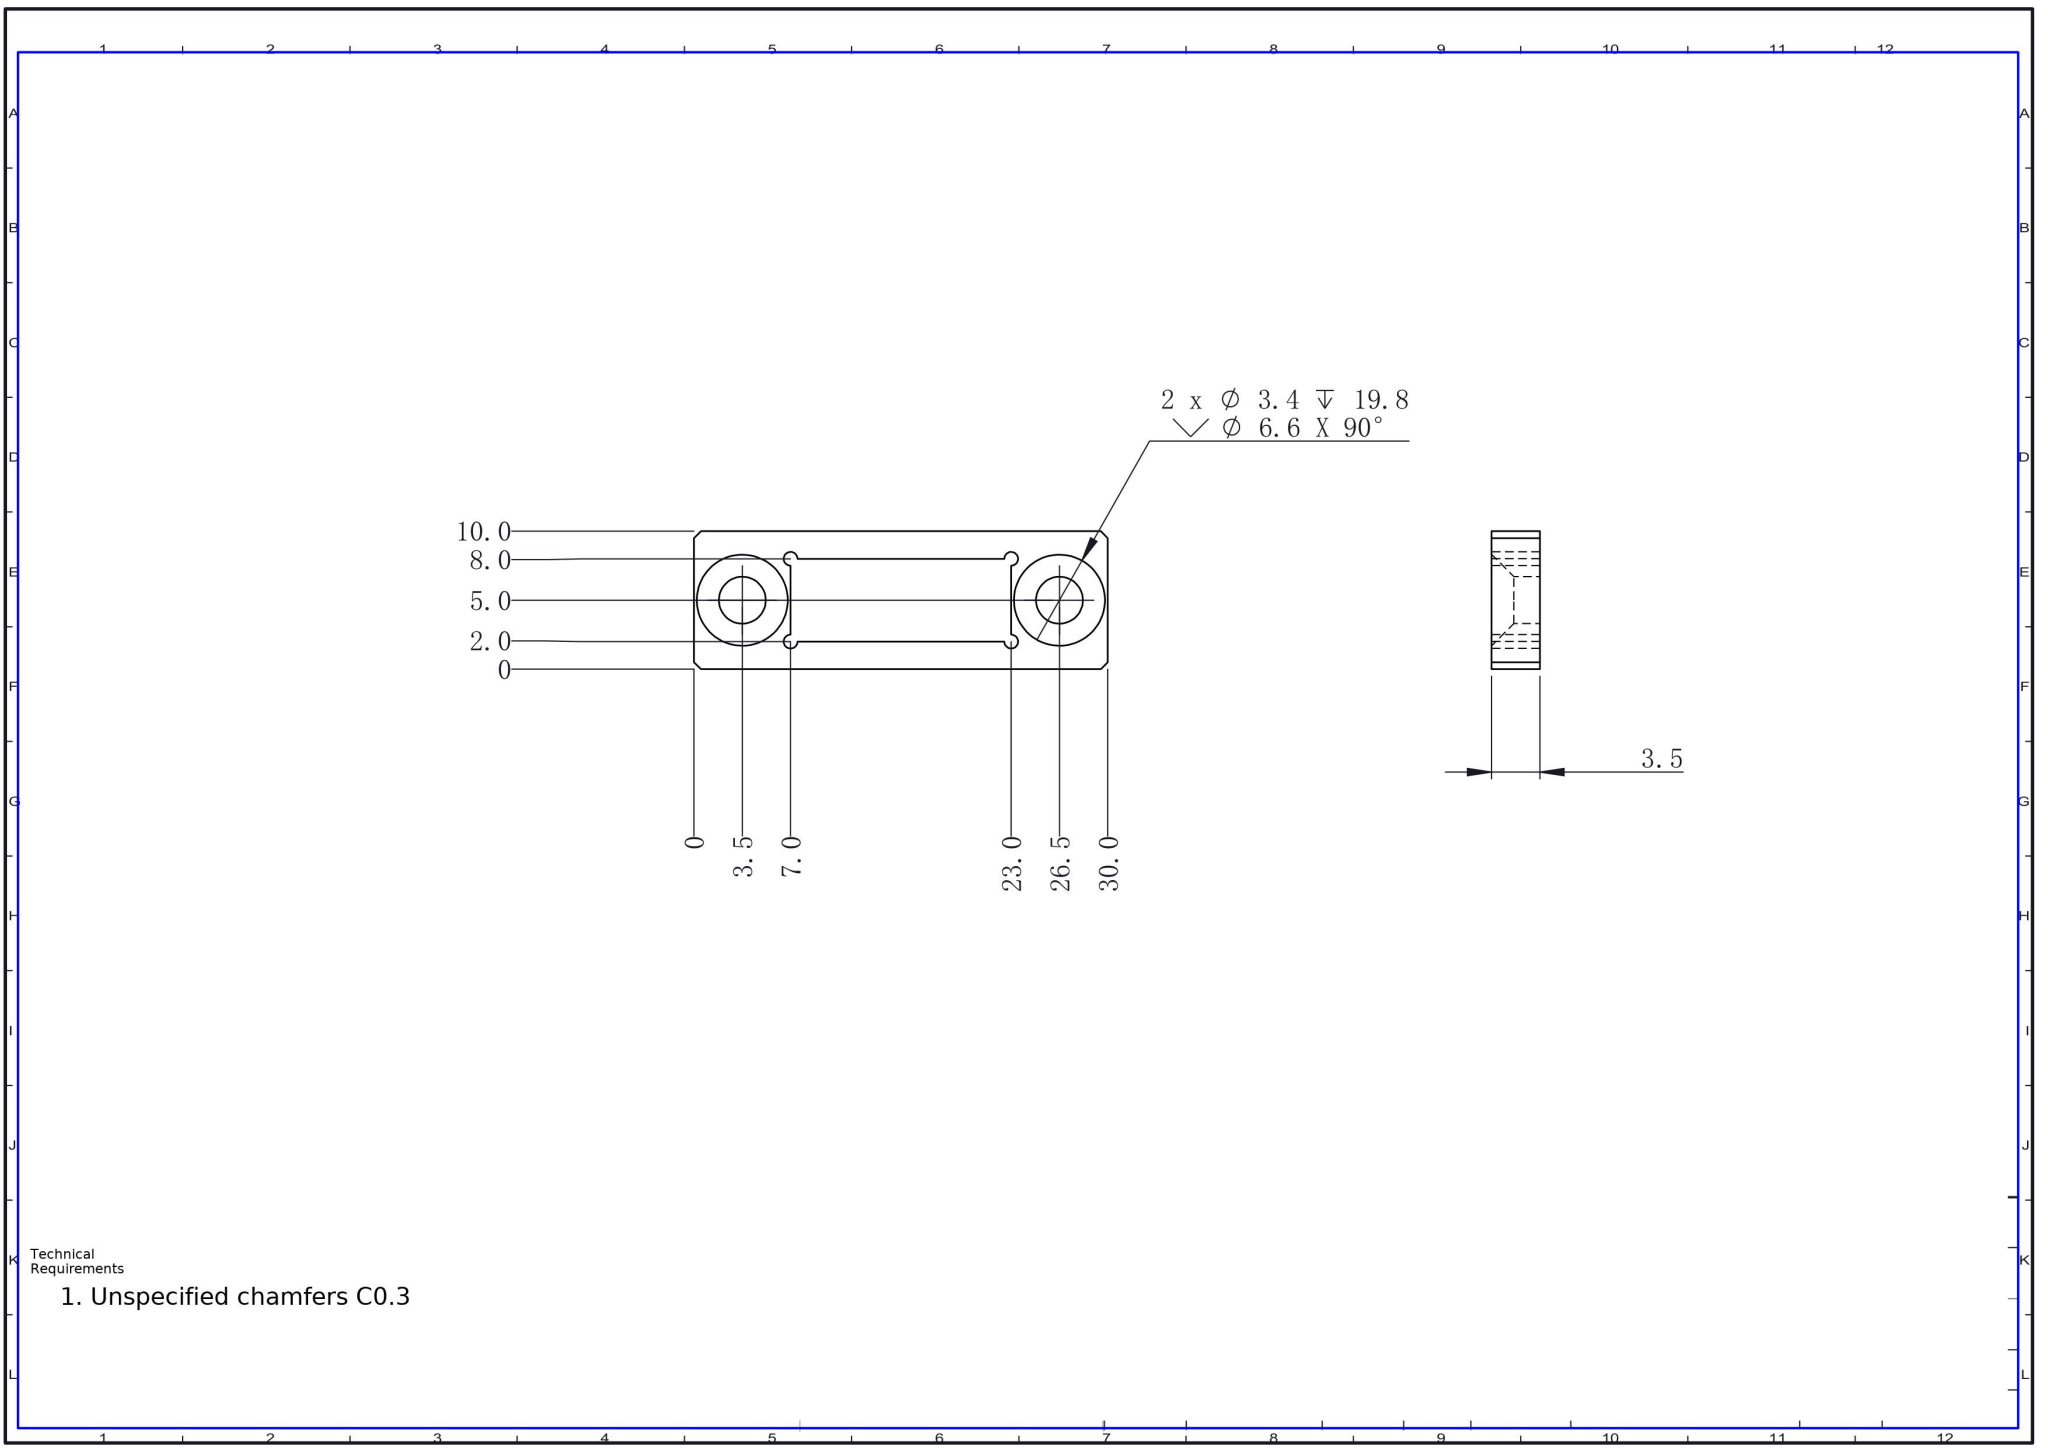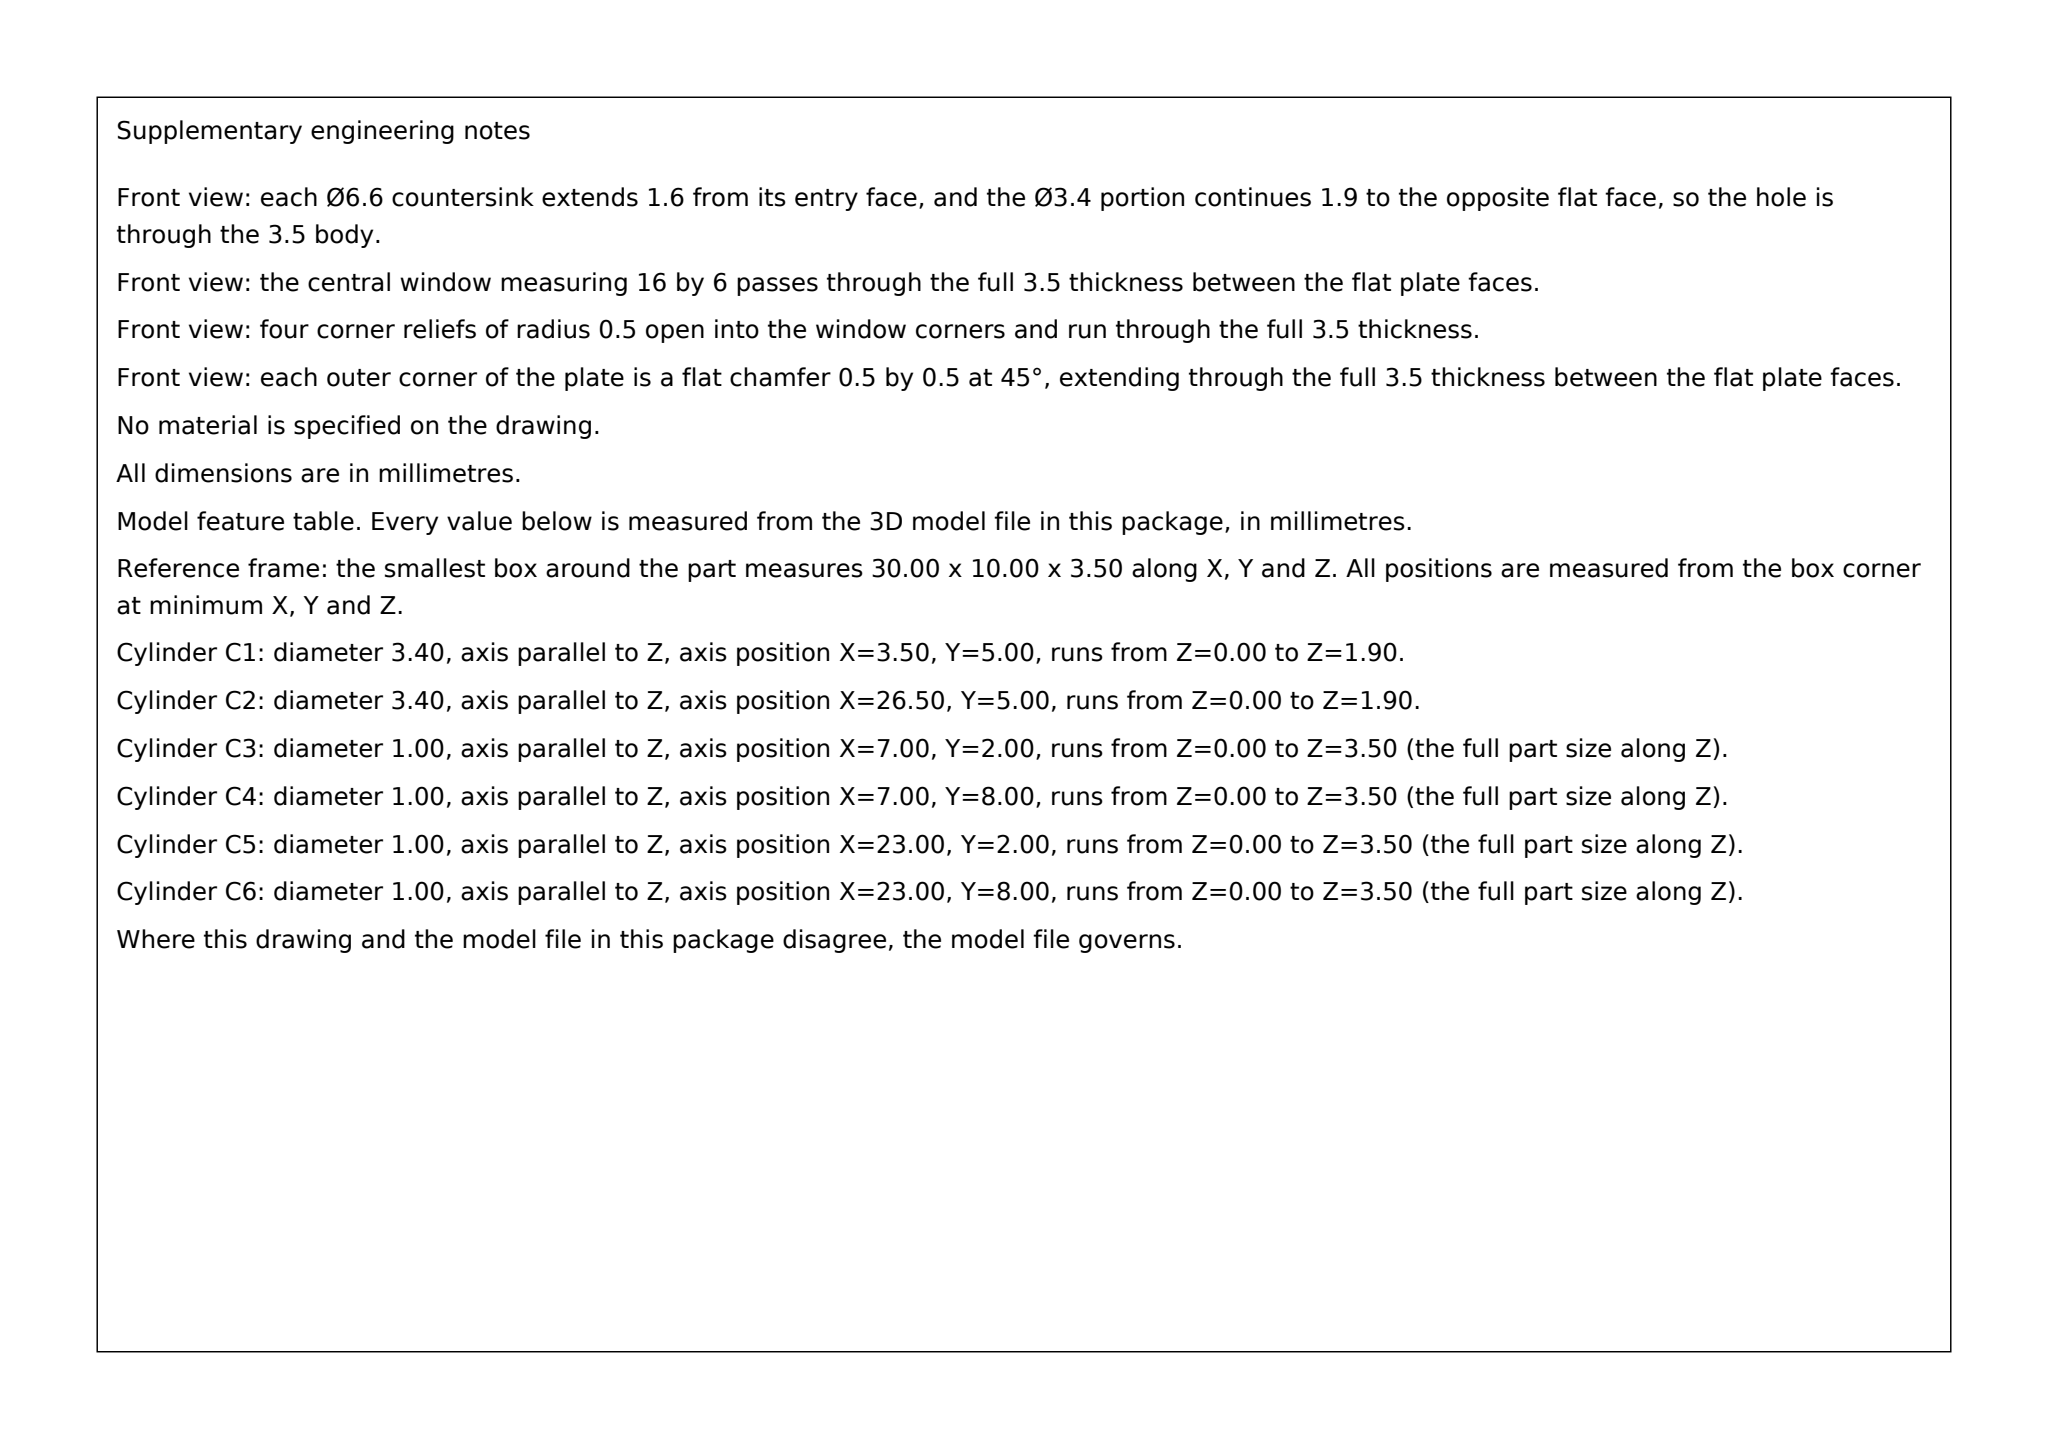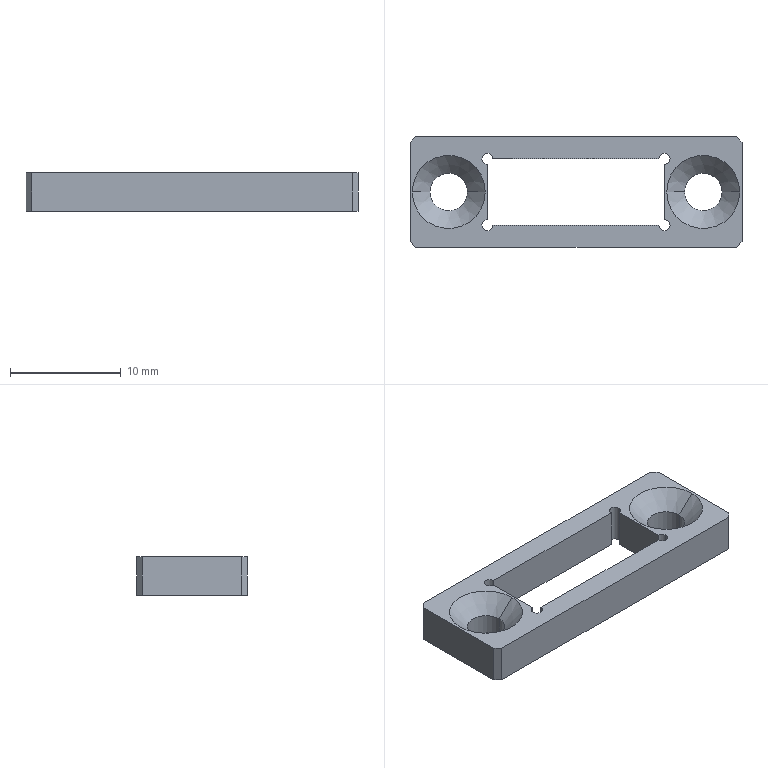Part | SolidWorks | mm | 1 solid | 28 faces | box 30 x 10 x 3.5 mm | volume 605 mm3 | plane 14 | cylinder 10 | cone 4 | commonest cylinder face diameters 1 x6 3.4 x4
Drawing notes:
2X Ø3.4 THRU ALL (NOT DP 19.8) | from the solid: Ø3.4 cyls at (3.5,5) & (26.5,5), 2 per hole x 1.9 deep from each face = 3.5 plate thk (thru)
CSK Ø6.6 X 90° NEAR & FAR SIDE, 4 PLCS | from the solid: cones[90.0, ref_dia 6.6] count = 4, i.e. both faces of each Ø3.4 hole
CTR SLOT 16 X 6 (X7.0-23.0, Y2.0-8.0) THRU ALL, 4X R0.5 | from the solid: planes x=7/23, y=2/8; corner Ø1.0 cyls length 3.5 = full plate thk
build123d program:
from build123d import *

# Parameters (mm, degrees)
SKETCH1_W                                          = 30
SKETCH1_H                                          = 10
SKETCH1_W_2                                        = 16
SKETCH1_H_2                                        = 6
BOSS_EXTRUDE1_DEPTH                                = 1.75
HOLE_SIZE_ACCORDING_TO_SLOTTED_COUNTER_D           = 3.4
HOLE_SIZE_ACCORDING_TO_SLOTTED_COUNTER_DEPTH       = 19.8
HOLE_SIZE_ACCORDING_TO_SLOTTED_COUNTER_CSINK_D     = 6.6
HOLE_SIZE_ACCORDING_TO_SLOTTED_COUNTER_CSINK_ANGLE = 90
HOLE_SIZE_ACCORDING_TO_SLOTTED_COUNTER_TIP         = 1.021
SKETCH6_R                                          = 0.5
CUT_EXTRUDE1_DEPTH                                 = 10
CHAMFER1_SIZE                                      = 0.5


with BuildPart() as part:
    # Sketch1 → Boss-Extrude1 (new, symmetric)
    with BuildSketch(Plane.XY):
        Rectangle(SKETCH1_W, SKETCH1_H)
        Rectangle(SKETCH1_W_2, SKETCH1_H_2, mode=Mode.SUBTRACT)
    extrude(amount=BOSS_EXTRUDE1_DEPTH, both=True)

    # Hole Size _According to_ Slotted Counter
    with Locations(Plane.XY.offset(1.75)):
        with Locations((-11.5, 0), (11.5, 0)):
            CounterSinkHole(HOLE_SIZE_ACCORDING_TO_SLOTTED_COUNTER_D / 2, HOLE_SIZE_ACCORDING_TO_SLOTTED_COUNTER_CSINK_D / 2, depth=HOLE_SIZE_ACCORDING_TO_SLOTTED_COUNTER_DEPTH, counter_sink_angle=HOLE_SIZE_ACCORDING_TO_SLOTTED_COUNTER_CSINK_ANGLE)
            with Locations((0, 0, -(HOLE_SIZE_ACCORDING_TO_SLOTTED_COUNTER_DEPTH + HOLE_SIZE_ACCORDING_TO_SLOTTED_COUNTER_TIP / 2))):  # 118° drill point
                Cone(0, HOLE_SIZE_ACCORDING_TO_SLOTTED_COUNTER_D / 2, HOLE_SIZE_ACCORDING_TO_SLOTTED_COUNTER_TIP, mode=Mode.SUBTRACT)

    # Sketch6 → Cut-Extrude1 (cut)
    with BuildSketch(Plane.XY.offset(1.75)):
        with Locations((-8, 3)):
            Circle(SKETCH6_R)
        with Locations((8, 3)):
            Circle(SKETCH6_R)
        with Locations((8, -3)):
            Circle(SKETCH6_R)
        with Locations((-8, -3)):
            Circle(SKETCH6_R)
    extrude(amount=-CUT_EXTRUDE1_DEPTH, mode=Mode.SUBTRACT)

    # Chamfer1
    chamfer1_edges = [part.edges().sort_by_distance(p)[0] for p in [
        (-15, 5, 0),
        (15, 5, 0),
        (15, -5, 0),
        (-15, -5, 0),
    ]]
    chamfer(chamfer1_edges, length=CHAMFER1_SIZE)


solid = part.part
STEP:
#1=CARTESIAN_POINT('',(8.5,-3.,-1.75));
#2=VERTEX_POINT('',#1);
#3=CARTESIAN_POINT('',(8.,-2.5,-1.75));
#4=VERTEX_POINT('',#3);
#5=CARTESIAN_POINT('',(8.,-3.,-1.75));
#6=DIRECTION('',(0.,0.,1.));
#7=DIRECTION('',(1.,0.,0.));
#8=AXIS2_PLACEMENT_3D('',#5,#6,#7);
#9=CIRCLE('',#8,0.5);
#10=EDGE_CURVE('',#2,#4,#9,.T.);
#11=ORIENTED_EDGE('',*,*,#10,.F.);
#12=CARTESIAN_POINT('',(8.5,-3.,1.75));
#13=VERTEX_POINT('',#12);
#14=CARTESIAN_POINT('',(8.5,-3.,-8.25));
#15=DIRECTION('',(0.,0.,1.));
#16=VECTOR('',#15,1000.);
#17=LINE('',#14,#16);
#18=EDGE_CURVE('',#2,#13,#17,.T.);
#19=ORIENTED_EDGE('',*,*,#18,.T.);
#20=CARTESIAN_POINT('',(8.,-2.5,1.75));
#21=VERTEX_POINT('',#20);
#22=CARTESIAN_POINT('',(8.,-3.,1.75));
#23=DIRECTION('',(0.,0.,1.));
#24=DIRECTION('',(1.,0.,0.));
#25=AXIS2_PLACEMENT_3D('',#22,#23,#24);
#26=CIRCLE('',#25,0.5);
#27=EDGE_CURVE('',#13,#21,#26,.T.);
#28=ORIENTED_EDGE('',*,*,#27,.T.);
#29=CARTESIAN_POINT('',(8.,-2.5,-8.25));
#30=DIRECTION('',(0.,0.,-1.));
#31=VECTOR('',#30,1000.);
#32=LINE('',#29,#31);
#33=EDGE_CURVE('',#21,#4,#32,.T.);
#34=ORIENTED_EDGE('',*,*,#33,.T.);
#35=EDGE_LOOP('',(#11,#19,#28,#34));
#36=FACE_OUTER_BOUND('',#35,.T.);
#37=CARTESIAN_POINT('',(8.,-3.,-8.25));
#38=DIRECTION('',(0.,0.,1.));
#39=DIRECTION('',(1.,0.,0.));
#40=AXIS2_PLACEMENT_3D('',#37,#38,#39);
#41=CYLINDRICAL_SURFACE('',#40,0.5);
#42=ADVANCED_FACE('',(#36),#41,.F.);
#43=CARTESIAN_POINT('',(8.5,3.,-1.75));
#44=VERTEX_POINT('',#43);
#45=CARTESIAN_POINT('',(7.5,3.,-1.75));
#46=VERTEX_POINT('',#45);
#47=CARTESIAN_POINT('',(8.,3.,-1.75));
#48=DIRECTION('',(0.,0.,1.));
#49=DIRECTION('',(1.,0.,0.));
#50=AXIS2_PLACEMENT_3D('',#47,#48,#49);
#51=CIRCLE('',#50,0.5);
#52=EDGE_CURVE('',#44,#46,#51,.T.);
#53=ORIENTED_EDGE('',*,*,#52,.F.);
#54=CARTESIAN_POINT('',(8.5,3.,1.75));
#55=VERTEX_POINT('',#54);
#56=CARTESIAN_POINT('',(8.5,3.,-8.25));
#57=DIRECTION('',(0.,0.,1.));
#58=VECTOR('',#57,1000.);
#59=LINE('',#56,#58);
#60=EDGE_CURVE('',#44,#55,#59,.T.);
#61=ORIENTED_EDGE('',*,*,#60,.T.);
#62=CARTESIAN_POINT('',(7.5,3.,1.75));
#63=VERTEX_POINT('',#62);
#64=CARTESIAN_POINT('',(8.,3.,1.75));
#65=DIRECTION('',(0.,0.,1.));
#66=DIRECTION('',(1.,0.,0.));
#67=AXIS2_PLACEMENT_3D('',#64,#65,#66);
#68=CIRCLE('',#67,0.5);
#69=EDGE_CURVE('',#55,#63,#68,.T.);
#70=ORIENTED_EDGE('',*,*,#69,.T.);
#71=CARTESIAN_POINT('',(7.5,3.,-8.25));
#72=DIRECTION('',(0.,0.,-1.));
#73=VECTOR('',#72,1000.);
#74=LINE('',#71,#73);
#75=EDGE_CURVE('',#63,#46,#74,.T.);
#76=ORIENTED_EDGE('',*,*,#75,.T.);
#77=EDGE_LOOP('',(#53,#61,#70,#76));
#78=FACE_OUTER_BOUND('',#77,.T.);
#79=CARTESIAN_POINT('',(8.,3.,-8.25));
#80=DIRECTION('',(0.,0.,1.));
#81=DIRECTION('',(1.,0.,0.));
#82=AXIS2_PLACEMENT_3D('',#79,#80,#81);
#83=CYLINDRICAL_SURFACE('',#82,0.5);
#84=ADVANCED_FACE('',(#78),#83,.F.);
#85=CARTESIAN_POINT('',(-13.2,0.,0.15));
#86=VERTEX_POINT('',#85);
#87=CARTESIAN_POINT('',(-9.8,0.,0.15));
#88=VERTEX_POINT('',#87);
#89=CARTESIAN_POINT('',(-11.5,0.,0.15));
#90=DIRECTION('',(0.,0.,1.));
#91=DIRECTION('',(1.,0.,0.));
#92=AXIS2_PLACEMENT_3D('',#89,#90,#91);
#93=CIRCLE('',#92,1.7);
#94=EDGE_CURVE('',#86,#88,#93,.T.);
#95=ORIENTED_EDGE('',*,*,#94,.F.);
#96=CARTESIAN_POINT('',(-14.8,0.,1.75));
#97=VERTEX_POINT('',#96);
#98=CARTESIAN_POINT('',(-14.8,0.,1.75));
#99=DIRECTION('',(-0.7071,0.,0.7071));
#100=VECTOR('',#99,1000.);
#101=LINE('',#98,#100);
#102=EDGE_CURVE('',#86,#97,#101,.T.);
#103=ORIENTED_EDGE('',*,*,#102,.T.);
#104=CARTESIAN_POINT('',(-8.2,0.,1.75));
#105=VERTEX_POINT('',#104);
#106=CARTESIAN_POINT('',(-11.5,0.,1.75));
#107=DIRECTION('',(0.,0.,1.));
#108=DIRECTION('',(1.,0.,0.));
#109=AXIS2_PLACEMENT_3D('',#106,#107,#108);
#110=CIRCLE('',#109,3.3);
#111=EDGE_CURVE('',#97,#105,#110,.T.);
#112=ORIENTED_EDGE('',*,*,#111,.T.);
#113=CARTESIAN_POINT('',(-8.2,0.,1.75));
#114=DIRECTION('',(0.7071,0.,0.7071));
#115=VECTOR('',#114,1000.);
#116=LINE('',#113,#115);
#117=EDGE_CURVE('',#88,#105,#116,.T.);
#118=ORIENTED_EDGE('',*,*,#117,.F.);
#119=EDGE_LOOP('',(#95,#103,#112,#118));
#120=FACE_OUTER_BOUND('',#119,.T.);
#121=CARTESIAN_POINT('',(-11.5,0.,1.75));
#122=DIRECTION('',(0.,0.,1.));
#123=DIRECTION('',(1.,0.,0.));
#124=AXIS2_PLACEMENT_3D('',#121,#122,#123);
#125=CONICAL_SURFACE('',#124,3.3,0.7854);
#126=ADVANCED_FACE('',(#120),#125,.F.);
#127=CARTESIAN_POINT('',(-13.2,0.,-1.75));
#128=VERTEX_POINT('',#127);
#129=CARTESIAN_POINT('',(-9.8,0.,-1.75));
#130=VERTEX_POINT('',#129);
#131=CARTESIAN_POINT('',(-11.5,0.,-1.75));
#132=DIRECTION('',(0.,0.,1.));
#133=DIRECTION('',(1.,0.,0.));
#134=AXIS2_PLACEMENT_3D('',#131,#132,#133);
#135=CIRCLE('',#134,1.7);
#136=EDGE_CURVE('',#128,#130,#135,.T.);
#137=ORIENTED_EDGE('',*,*,#136,.F.);
#138=CARTESIAN_POINT('',(-13.2,0.,1.75));
#139=DIRECTION('',(0.,0.,1.));
#140=VECTOR('',#139,1000.);
#141=LINE('',#138,#140);
#142=EDGE_CURVE('',#128,#86,#141,.T.);
#143=ORIENTED_EDGE('',*,*,#142,.T.);
#144=ORIENTED_EDGE('',*,*,#94,.T.);
#145=CARTESIAN_POINT('',(-9.8,0.,1.75));
#146=DIRECTION('',(0.,0.,1.));
#147=VECTOR('',#146,1000.);
#148=LINE('',#145,#147);
#149=EDGE_CURVE('',#130,#88,#148,.T.);
#150=ORIENTED_EDGE('',*,*,#149,.F.);
#151=EDGE_LOOP('',(#137,#143,#144,#150));
#152=FACE_OUTER_BOUND('',#151,.T.);
#153=CARTESIAN_POINT('',(-11.5,0.,1.75));
#154=DIRECTION('',(0.,0.,1.));
#155=DIRECTION('',(1.,0.,0.));
#156=AXIS2_PLACEMENT_3D('',#153,#154,#155);
#157=CYLINDRICAL_SURFACE('',#156,1.7);
#158=ADVANCED_FACE('',(#152),#157,.F.);
#159=CARTESIAN_POINT('',(9.8,0.,0.15));
#160=VERTEX_POINT('',#159);
#161=CARTESIAN_POINT('',(13.2,0.,0.15));
#162=VERTEX_POINT('',#161);
#163=CARTESIAN_POINT('',(11.5,0.,0.15));
#164=DIRECTION('',(0.,0.,1.));
#165=DIRECTION('',(1.,0.,0.));
#166=AXIS2_PLACEMENT_3D('',#163,#164,#165);
#167=CIRCLE('',#166,1.7);
#168=EDGE_CURVE('',#160,#162,#167,.T.);
#169=ORIENTED_EDGE('',*,*,#168,.F.);
#170=CARTESIAN_POINT('',(8.2,0.,1.75));
#171=VERTEX_POINT('',#170);
#172=CARTESIAN_POINT('',(8.2,0.,1.75));
#173=DIRECTION('',(-0.7071,0.,0.7071));
#174=VECTOR('',#173,1000.);
#175=LINE('',#172,#174);
#176=EDGE_CURVE('',#160,#171,#175,.T.);
#177=ORIENTED_EDGE('',*,*,#176,.T.);
#178=CARTESIAN_POINT('',(14.8,0.,1.75));
#179=VERTEX_POINT('',#178);
#180=CARTESIAN_POINT('',(11.5,0.,1.75));
#181=DIRECTION('',(0.,0.,1.));
#182=DIRECTION('',(1.,0.,0.));
#183=AXIS2_PLACEMENT_3D('',#180,#181,#182);
#184=CIRCLE('',#183,3.3);
#185=EDGE_CURVE('',#171,#179,#184,.T.);
#186=ORIENTED_EDGE('',*,*,#185,.T.);
#187=CARTESIAN_POINT('',(14.8,0.,1.75));
#188=DIRECTION('',(0.7071,0.,0.7071));
#189=VECTOR('',#188,1000.);
#190=LINE('',#187,#189);
#191=EDGE_CURVE('',#162,#179,#190,.T.);
#192=ORIENTED_EDGE('',*,*,#191,.F.);
#193=EDGE_LOOP('',(#169,#177,#186,#192));
#194=FACE_OUTER_BOUND('',#193,.T.);
#195=CARTESIAN_POINT('',(11.5,0.,1.75));
#196=DIRECTION('',(0.,0.,1.));
#197=DIRECTION('',(1.,0.,0.));
#198=AXIS2_PLACEMENT_3D('',#195,#196,#197);
#199=CONICAL_SURFACE('',#198,3.3,0.7854);
#200=ADVANCED_FACE('',(#194),#199,.F.);
#201=CARTESIAN_POINT('',(9.8,0.,-1.75));
#202=VERTEX_POINT('',#201);
#203=CARTESIAN_POINT('',(13.2,0.,-1.75));
#204=VERTEX_POINT('',#203);
#205=CARTESIAN_POINT('',(11.5,0.,-1.75));
#206=DIRECTION('',(0.,0.,1.));
#207=DIRECTION('',(1.,0.,0.));
#208=AXIS2_PLACEMENT_3D('',#205,#206,#207);
#209=CIRCLE('',#208,1.7);
#210=EDGE_CURVE('',#202,#204,#209,.T.);
#211=ORIENTED_EDGE('',*,*,#210,.F.);
#212=CARTESIAN_POINT('',(9.8,0.,1.75));
#213=DIRECTION('',(0.,0.,1.));
#214=VECTOR('',#213,1000.);
#215=LINE('',#212,#214);
#216=EDGE_CURVE('',#202,#160,#215,.T.);
#217=ORIENTED_EDGE('',*,*,#216,.T.);
#218=ORIENTED_EDGE('',*,*,#168,.T.);
#219=CARTESIAN_POINT('',(13.2,0.,1.75));
#220=DIRECTION('',(0.,0.,1.));
#221=VECTOR('',#220,1000.);
#222=LINE('',#219,#221);
#223=EDGE_CURVE('',#204,#162,#222,.T.);
#224=ORIENTED_EDGE('',*,*,#223,.F.);
#225=EDGE_LOOP('',(#211,#217,#218,#224));
#226=FACE_OUTER_BOUND('',#225,.T.);
#227=CARTESIAN_POINT('',(11.5,0.,1.75));
#228=DIRECTION('',(0.,0.,1.));
#229=DIRECTION('',(1.,0.,0.));
#230=AXIS2_PLACEMENT_3D('',#227,#228,#229);
#231=CYLINDRICAL_SURFACE('',#230,1.7);
#232=ADVANCED_FACE('',(#226),#231,.F.);
#233=CARTESIAN_POINT('',(-8.,-2.5,1.75));
#234=VERTEX_POINT('',#233);
#235=CARTESIAN_POINT('',(-7.5,-3.,1.75));
#236=VERTEX_POINT('',#235);
#237=CARTESIAN_POINT('',(-8.,-3.,1.75));
#238=DIRECTION('',(0.,0.,1.));
#239=DIRECTION('',(1.,0.,0.));
#240=AXIS2_PLACEMENT_3D('',#237,#238,#239);
#241=CIRCLE('',#240,0.5);
#242=EDGE_CURVE('',#234,#236,#241,.T.);
#243=ORIENTED_EDGE('',*,*,#242,.F.);
#244=CARTESIAN_POINT('',(-8.,2.5,1.75));
#245=VERTEX_POINT('',#244);
#246=CARTESIAN_POINT('',(-8.,3.,1.75));
#247=DIRECTION('',(-0.,-1.,0.));
#248=VECTOR('',#247,1000.);
#249=LINE('',#246,#248);
#250=EDGE_CURVE('',#245,#234,#249,.T.);
#251=ORIENTED_EDGE('',*,*,#250,.F.);
#252=CARTESIAN_POINT('',(-7.5,3.,1.75));
#253=VERTEX_POINT('',#252);
#254=CARTESIAN_POINT('',(-8.,3.,1.75));
#255=DIRECTION('',(0.,0.,1.));
#256=DIRECTION('',(1.,0.,0.));
#257=AXIS2_PLACEMENT_3D('',#254,#255,#256);
#258=CIRCLE('',#257,0.5);
#259=EDGE_CURVE('',#253,#245,#258,.T.);
#260=ORIENTED_EDGE('',*,*,#259,.F.);
#261=CARTESIAN_POINT('',(-8.,3.,1.75));
#262=DIRECTION('',(-1.,-0.,0.));
#263=VECTOR('',#262,1000.);
#264=LINE('',#261,#263);
#265=EDGE_CURVE('',#63,#253,#264,.T.);
#266=ORIENTED_EDGE('',*,*,#265,.F.);
#267=ORIENTED_EDGE('',*,*,#69,.F.);
#268=CARTESIAN_POINT('',(8.,2.5,1.75));
#269=VERTEX_POINT('',#268);
#270=CARTESIAN_POINT('',(8.,3.,1.75));
#271=DIRECTION('',(0.,0.,1.));
#272=DIRECTION('',(1.,0.,0.));
#273=AXIS2_PLACEMENT_3D('',#270,#271,#272);
#274=CIRCLE('',#273,0.5);
#275=EDGE_CURVE('',#269,#55,#274,.T.);
#276=ORIENTED_EDGE('',*,*,#275,.F.);
#277=CARTESIAN_POINT('',(8.,3.,1.75));
#278=DIRECTION('',(-0.,1.,0.));
#279=VECTOR('',#278,1000.);
#280=LINE('',#277,#279);
#281=EDGE_CURVE('',#21,#269,#280,.T.);
#282=ORIENTED_EDGE('',*,*,#281,.F.);
#283=ORIENTED_EDGE('',*,*,#27,.F.);
#284=CARTESIAN_POINT('',(7.5,-3.,1.75));
#285=VERTEX_POINT('',#284);
#286=CARTESIAN_POINT('',(8.,-3.,1.75));
#287=DIRECTION('',(0.,0.,1.));
#288=DIRECTION('',(1.,0.,0.));
#289=AXIS2_PLACEMENT_3D('',#286,#287,#288);
#290=CIRCLE('',#289,0.5);
#291=EDGE_CURVE('',#285,#13,#290,.T.);
#292=ORIENTED_EDGE('',*,*,#291,.F.);
#293=CARTESIAN_POINT('',(-8.,-3.,1.75));
#294=DIRECTION('',(1.,0.,0.));
#295=VECTOR('',#294,1000.);
#296=LINE('',#293,#295);
#297=EDGE_CURVE('',#236,#285,#296,.T.);
#298=ORIENTED_EDGE('',*,*,#297,.F.);
#299=EDGE_LOOP('',(#243,#251,#260,#266,#267,#276,#282,#283,#292,#298));
#300=FACE_BOUND('',#299,.T.);
#301=CARTESIAN_POINT('',(-11.5,0.,1.75));
#302=DIRECTION('',(0.,0.,1.));
#303=DIRECTION('',(1.,0.,0.));
#304=AXIS2_PLACEMENT_3D('',#301,#302,#303);
#305=CIRCLE('',#304,3.3);
#306=EDGE_CURVE('',#105,#97,#305,.T.);
#307=ORIENTED_EDGE('',*,*,#306,.F.);
#308=ORIENTED_EDGE('',*,*,#111,.F.);
#309=EDGE_LOOP('',(#307,#308));
#310=FACE_BOUND('',#309,.T.);
#311=CARTESIAN_POINT('',(11.5,0.,1.75));
#312=DIRECTION('',(0.,0.,1.));
#313=DIRECTION('',(1.,0.,0.));
#314=AXIS2_PLACEMENT_3D('',#311,#312,#313);
#315=CIRCLE('',#314,3.3);
#316=EDGE_CURVE('',#179,#171,#315,.T.);
#317=ORIENTED_EDGE('',*,*,#316,.F.);
#318=ORIENTED_EDGE('',*,*,#185,.F.);
#319=EDGE_LOOP('',(#317,#318));
#320=FACE_BOUND('',#319,.T.);
#321=CARTESIAN_POINT('',(14.5,5.,1.75));
#322=VERTEX_POINT('',#321);
#323=CARTESIAN_POINT('',(-14.5,5.,1.75));
#324=VERTEX_POINT('',#323);
#325=CARTESIAN_POINT('',(-15.,5.,1.75));
#326=DIRECTION('',(-1.,-0.,0.));
#327=VECTOR('',#326,1000.);
#328=LINE('',#325,#327);
#329=EDGE_CURVE('',#322,#324,#328,.T.);
#330=ORIENTED_EDGE('',*,*,#329,.T.);
#331=CARTESIAN_POINT('',(-15.,4.5,1.75));
#332=VERTEX_POINT('',#331);
#333=CARTESIAN_POINT('',(-9.75,9.75,1.75));
#334=DIRECTION('',(-0.7071,-0.7071,0.));
#335=VECTOR('',#334,1000.);
#336=LINE('',#333,#335);
#337=EDGE_CURVE('',#324,#332,#336,.T.);
#338=ORIENTED_EDGE('',*,*,#337,.T.);
#339=CARTESIAN_POINT('',(-15.,-4.5,1.75));
#340=VERTEX_POINT('',#339);
#341=CARTESIAN_POINT('',(-15.,5.,1.75));
#342=DIRECTION('',(0.,-1.,0.));
#343=VECTOR('',#342,1000.);
#344=LINE('',#341,#343);
#345=EDGE_CURVE('',#332,#340,#344,.T.);
#346=ORIENTED_EDGE('',*,*,#345,.T.);
#347=CARTESIAN_POINT('',(-14.5,-5.,1.75));
#348=VERTEX_POINT('',#347);
#349=CARTESIAN_POINT('',(-9.75,-9.75,1.75));
#350=DIRECTION('',(0.7071,-0.7071,0.));
#351=VECTOR('',#350,1000.);
#352=LINE('',#349,#351);
#353=EDGE_CURVE('',#340,#348,#352,.T.);
#354=ORIENTED_EDGE('',*,*,#353,.T.);
#355=CARTESIAN_POINT('',(14.5,-5.,1.75));
#356=VERTEX_POINT('',#355);
#357=CARTESIAN_POINT('',(-15.,-5.,1.75));
#358=DIRECTION('',(1.,0.,0.));
#359=VECTOR('',#358,1000.);
#360=LINE('',#357,#359);
#361=EDGE_CURVE('',#348,#356,#360,.T.);
#362=ORIENTED_EDGE('',*,*,#361,.T.);
#363=CARTESIAN_POINT('',(15.,-4.5,1.75));
#364=VERTEX_POINT('',#363);
#365=CARTESIAN_POINT('',(9.75,-9.75,1.75));
#366=DIRECTION('',(0.7071,0.7071,0.));
#367=VECTOR('',#366,1000.);
#368=LINE('',#365,#367);
#369=EDGE_CURVE('',#356,#364,#368,.T.);
#370=ORIENTED_EDGE('',*,*,#369,.T.);
#371=CARTESIAN_POINT('',(15.,4.5,1.75));
#372=VERTEX_POINT('',#371);
#373=CARTESIAN_POINT('',(15.,5.,1.75));
#374=DIRECTION('',(0.,1.,0.));
#375=VECTOR('',#374,1000.);
#376=LINE('',#373,#375);
#377=EDGE_CURVE('',#364,#372,#376,.T.);
#378=ORIENTED_EDGE('',*,*,#377,.T.);
#379=CARTESIAN_POINT('',(9.75,9.75,1.75));
#380=DIRECTION('',(-0.7071,0.7071,0.));
#381=VECTOR('',#380,1000.);
#382=LINE('',#379,#381);
#383=EDGE_CURVE('',#372,#322,#382,.T.);
#384=ORIENTED_EDGE('',*,*,#383,.T.);
#385=EDGE_LOOP('',(#330,#338,#346,#354,#362,#370,#378,#384));
#386=FACE_OUTER_BOUND('',#385,.T.);
#387=CARTESIAN_POINT('',(0.,0.,1.75));
#388=DIRECTION('',(0.,0.,1.));
#389=DIRECTION('',(1.,0.,0.));
#390=AXIS2_PLACEMENT_3D('',#387,#388,#389);
#391=PLANE('',#390);
#392=ADVANCED_FACE('',(#300,#310,#320,#386),#391,.T.);
#393=CARTESIAN_POINT('',(-11.5,0.,-1.75));
#394=DIRECTION('',(0.,0.,1.));
#395=DIRECTION('',(1.,0.,0.));
#396=AXIS2_PLACEMENT_3D('',#393,#394,#395);
#397=CIRCLE('',#396,1.7);
#398=EDGE_CURVE('',#130,#128,#397,.T.);
#399=ORIENTED_EDGE('',*,*,#398,.T.);
#400=ORIENTED_EDGE('',*,*,#136,.T.);
#401=EDGE_LOOP('',(#399,#400));
#402=FACE_BOUND('',#401,.T.);
#403=CARTESIAN_POINT('',(11.5,0.,-1.75));
#404=DIRECTION('',(0.,0.,1.));
#405=DIRECTION('',(1.,0.,0.));
#406=AXIS2_PLACEMENT_3D('',#403,#404,#405);
#407=CIRCLE('',#406,1.7);
#408=EDGE_CURVE('',#204,#202,#407,.T.);
#409=ORIENTED_EDGE('',*,*,#408,.T.);
#410=ORIENTED_EDGE('',*,*,#210,.T.);
#411=EDGE_LOOP('',(#409,#410));
#412=FACE_BOUND('',#411,.T.);
#413=CARTESIAN_POINT('',(-15.,4.5,-1.75));
#414=VERTEX_POINT('',#413);
#415=CARTESIAN_POINT('',(-15.,-4.5,-1.75));
#416=VERTEX_POINT('',#415);
#417=CARTESIAN_POINT('',(-15.,5.,-1.75));
#418=DIRECTION('',(0.,-1.,0.));
#419=VECTOR('',#418,1000.);
#420=LINE('',#417,#419);
#421=EDGE_CURVE('',#414,#416,#420,.T.);
#422=ORIENTED_EDGE('',*,*,#421,.F.);
#423=CARTESIAN_POINT('',(-14.5,5.,-1.75));
#424=VERTEX_POINT('',#423);
#425=CARTESIAN_POINT('',(-15.,4.5,-1.75));
#426=DIRECTION('',(0.7071,0.7071,0.));
#427=VECTOR('',#426,1000.);
#428=LINE('',#425,#427);
#429=EDGE_CURVE('',#414,#424,#428,.T.);
#430=ORIENTED_EDGE('',*,*,#429,.T.);
#431=CARTESIAN_POINT('',(14.5,5.,-1.75));
#432=VERTEX_POINT('',#431);
#433=CARTESIAN_POINT('',(-15.,5.,-1.75));
#434=DIRECTION('',(-1.,-0.,0.));
#435=VECTOR('',#434,1000.);
#436=LINE('',#433,#435);
#437=EDGE_CURVE('',#432,#424,#436,.T.);
#438=ORIENTED_EDGE('',*,*,#437,.F.);
#439=CARTESIAN_POINT('',(15.,4.5,-1.75));
#440=VERTEX_POINT('',#439);
#441=CARTESIAN_POINT('',(14.5,5.,-1.75));
#442=DIRECTION('',(0.7071,-0.7071,0.));
#443=VECTOR('',#442,1000.);
#444=LINE('',#441,#443);
#445=EDGE_CURVE('',#432,#440,#444,.T.);
#446=ORIENTED_EDGE('',*,*,#445,.T.);
#447=CARTESIAN_POINT('',(15.,-4.5,-1.75));
#448=VERTEX_POINT('',#447);
#449=CARTESIAN_POINT('',(15.,5.,-1.75));
#450=DIRECTION('',(0.,1.,0.));
#451=VECTOR('',#450,1000.);
#452=LINE('',#449,#451);
#453=EDGE_CURVE('',#448,#440,#452,.T.);
#454=ORIENTED_EDGE('',*,*,#453,.F.);
#455=CARTESIAN_POINT('',(14.5,-5.,-1.75));
#456=VERTEX_POINT('',#455);
#457=CARTESIAN_POINT('',(15.,-4.5,-1.75));
#458=DIRECTION('',(-0.7071,-0.7071,0.));
#459=VECTOR('',#458,1000.);
#460=LINE('',#457,#459);
#461=EDGE_CURVE('',#448,#456,#460,.T.);
#462=ORIENTED_EDGE('',*,*,#461,.T.);
#463=CARTESIAN_POINT('',(-14.5,-5.,-1.75));
#464=VERTEX_POINT('',#463);
#465=CARTESIAN_POINT('',(-15.,-5.,-1.75));
#466=DIRECTION('',(1.,0.,0.));
#467=VECTOR('',#466,1000.);
#468=LINE('',#465,#467);
#469=EDGE_CURVE('',#464,#456,#468,.T.);
#470=ORIENTED_EDGE('',*,*,#469,.F.);
#471=CARTESIAN_POINT('',(-14.5,-5.,-1.75));
#472=DIRECTION('',(-0.7071,0.7071,0.));
#473=VECTOR('',#472,1000.);
#474=LINE('',#471,#473);
#475=EDGE_CURVE('',#464,#416,#474,.T.);
#476=ORIENTED_EDGE('',*,*,#475,.T.);
#477=EDGE_LOOP('',(#422,#430,#438,#446,#454,#462,#470,#476));
#478=FACE_OUTER_BOUND('',#477,.T.);
#479=CARTESIAN_POINT('',(-8.,2.5,-1.75));
#480=VERTEX_POINT('',#479);
#481=CARTESIAN_POINT('',(-8.,-2.5,-1.75));
#482=VERTEX_POINT('',#481);
#483=CARTESIAN_POINT('',(-8.,3.,-1.75));
#484=DIRECTION('',(-0.,-1.,0.));
#485=VECTOR('',#484,1000.);
#486=LINE('',#483,#485);
#487=EDGE_CURVE('',#480,#482,#486,.T.);
#488=ORIENTED_EDGE('',*,*,#487,.T.);
#489=CARTESIAN_POINT('',(-7.5,-3.,-1.75));
#490=VERTEX_POINT('',#489);
#491=CARTESIAN_POINT('',(-8.,-3.,-1.75));
#492=DIRECTION('',(0.,0.,1.));
#493=DIRECTION('',(1.,0.,0.));
#494=AXIS2_PLACEMENT_3D('',#491,#492,#493);
#495=CIRCLE('',#494,0.5);
#496=EDGE_CURVE('',#482,#490,#495,.T.);
#497=ORIENTED_EDGE('',*,*,#496,.T.);
#498=CARTESIAN_POINT('',(7.5,-3.,-1.75));
#499=VERTEX_POINT('',#498);
#500=CARTESIAN_POINT('',(-8.,-3.,-1.75));
#501=DIRECTION('',(1.,0.,0.));
#502=VECTOR('',#501,1000.);
#503=LINE('',#500,#502);
#504=EDGE_CURVE('',#490,#499,#503,.T.);
#505=ORIENTED_EDGE('',*,*,#504,.T.);
#506=CARTESIAN_POINT('',(8.,-3.,-1.75));
#507=DIRECTION('',(0.,0.,1.));
#508=DIRECTION('',(1.,0.,0.));
#509=AXIS2_PLACEMENT_3D('',#506,#507,#508);
#510=CIRCLE('',#509,0.5);
#511=EDGE_CURVE('',#499,#2,#510,.T.);
#512=ORIENTED_EDGE('',*,*,#511,.T.);
#513=ORIENTED_EDGE('',*,*,#10,.T.);
#514=CARTESIAN_POINT('',(8.,2.5,-1.75));
#515=VERTEX_POINT('',#514);
#516=CARTESIAN_POINT('',(8.,3.,-1.75));
#517=DIRECTION('',(-0.,1.,0.));
#518=VECTOR('',#517,1000.);
#519=LINE('',#516,#518);
#520=EDGE_CURVE('',#4,#515,#519,.T.);
#521=ORIENTED_EDGE('',*,*,#520,.T.);
#522=CARTESIAN_POINT('',(8.,3.,-1.75));
#523=DIRECTION('',(0.,0.,1.));
#524=DIRECTION('',(1.,0.,0.));
#525=AXIS2_PLACEMENT_3D('',#522,#523,#524);
#526=CIRCLE('',#525,0.5);
#527=EDGE_CURVE('',#515,#44,#526,.T.);
#528=ORIENTED_EDGE('',*,*,#527,.T.);
#529=ORIENTED_EDGE('',*,*,#52,.T.);
#530=CARTESIAN_POINT('',(-7.5,3.,-1.75));
#531=VERTEX_POINT('',#530);
#532=CARTESIAN_POINT('',(-8.,3.,-1.75));
#533=DIRECTION('',(-1.,-0.,0.));
#534=VECTOR('',#533,1000.);
#535=LINE('',#532,#534);
#536=EDGE_CURVE('',#46,#531,#535,.T.);
#537=ORIENTED_EDGE('',*,*,#536,.T.);
#538=CARTESIAN_POINT('',(-8.,3.,-1.75));
#539=DIRECTION('',(0.,0.,1.));
#540=DIRECTION('',(1.,0.,0.));
#541=AXIS2_PLACEMENT_3D('',#538,#539,#540);
#542=CIRCLE('',#541,0.5);
#543=EDGE_CURVE('',#531,#480,#542,.T.);
#544=ORIENTED_EDGE('',*,*,#543,.T.);
#545=EDGE_LOOP('',(#488,#497,#505,#512,#513,#521,#528,#529,#537,#544));
#546=FACE_BOUND('',#545,.T.);
#547=CARTESIAN_POINT('',(0.,0.,-1.75));
#548=DIRECTION('',(0.,0.,1.));
#549=DIRECTION('',(1.,0.,0.));
#550=AXIS2_PLACEMENT_3D('',#547,#548,#549);
#551=PLANE('',#550);
#552=ADVANCED_FACE('',(#402,#412,#478,#546),#551,.F.);
#553=ORIENTED_EDGE('',*,*,#345,.F.);
#554=CARTESIAN_POINT('',(-15.,4.5,1.75));
#555=DIRECTION('',(0.,0.,-1.));
#556=VECTOR('',#555,1000.);
#557=LINE('',#554,#556);
#558=EDGE_CURVE('',#332,#414,#557,.T.);
#559=ORIENTED_EDGE('',*,*,#558,.T.);
#560=ORIENTED_EDGE('',*,*,#421,.T.);
#561=CARTESIAN_POINT('',(-15.,-4.5,1.75));
#562=DIRECTION('',(0.,0.,1.));
#563=VECTOR('',#562,1000.);
#564=LINE('',#561,#563);
#565=EDGE_CURVE('',#416,#340,#564,.T.);
#566=ORIENTED_EDGE('',*,*,#565,.T.);
#567=EDGE_LOOP('',(#553,#559,#560,#566));
#568=FACE_OUTER_BOUND('',#567,.T.);
#569=CARTESIAN_POINT('',(-15.,5.,1.75));
#570=DIRECTION('',(1.,0.,0.));
#571=DIRECTION('',(0.,0.,-1.));
#572=AXIS2_PLACEMENT_3D('',#569,#570,#571);
#573=PLANE('',#572);
#574=ADVANCED_FACE('',(#568),#573,.F.);
#575=ORIENTED_EDGE('',*,*,#361,.F.);
#576=CARTESIAN_POINT('',(-14.5,-5.,1.75));
#577=DIRECTION('',(0.,0.,-1.));
#578=VECTOR('',#577,1000.);
#579=LINE('',#576,#578);
#580=EDGE_CURVE('',#348,#464,#579,.T.);
#581=ORIENTED_EDGE('',*,*,#580,.T.);
#582=ORIENTED_EDGE('',*,*,#469,.T.);
#583=CARTESIAN_POINT('',(14.5,-5.,1.75));
#584=DIRECTION('',(0.,0.,1.));
#585=VECTOR('',#584,1000.);
#586=LINE('',#583,#585);
#587=EDGE_CURVE('',#456,#356,#586,.T.);
#588=ORIENTED_EDGE('',*,*,#587,.T.);
#589=EDGE_LOOP('',(#575,#581,#582,#588));
#590=FACE_OUTER_BOUND('',#589,.T.);
#591=CARTESIAN_POINT('',(-15.,-5.,1.75));
#592=DIRECTION('',(-0.,1.,0.));
#593=DIRECTION('',(-1.,-0.,0.));
#594=AXIS2_PLACEMENT_3D('',#591,#592,#593);
#595=PLANE('',#594);
#596=ADVANCED_FACE('',(#590),#595,.F.);
#597=ORIENTED_EDGE('',*,*,#377,.F.);
#598=CARTESIAN_POINT('',(15.,-4.5,1.75));
#599=DIRECTION('',(0.,0.,-1.));
#600=VECTOR('',#599,1000.);
#601=LINE('',#598,#600);
#602=EDGE_CURVE('',#364,#448,#601,.T.);
#603=ORIENTED_EDGE('',*,*,#602,.T.);
#604=ORIENTED_EDGE('',*,*,#453,.T.);
#605=CARTESIAN_POINT('',(15.,4.5,1.75));
#606=DIRECTION('',(0.,0.,1.));
#607=VECTOR('',#606,1000.);
#608=LINE('',#605,#607);
#609=EDGE_CURVE('',#440,#372,#608,.T.);
#610=ORIENTED_EDGE('',*,*,#609,.T.);
#611=EDGE_LOOP('',(#597,#603,#604,#610));
#612=FACE_OUTER_BOUND('',#611,.T.);
#613=CARTESIAN_POINT('',(15.,5.,1.75));
#614=DIRECTION('',(-1.,0.,0.));
#615=DIRECTION('',(0.,0.,1.));
#616=AXIS2_PLACEMENT_3D('',#613,#614,#615);
#617=PLANE('',#616);
#618=ADVANCED_FACE('',(#612),#617,.F.);
#619=ORIENTED_EDGE('',*,*,#437,.T.);
#620=CARTESIAN_POINT('',(-14.5,5.,1.75));
#621=DIRECTION('',(0.,0.,1.));
#622=VECTOR('',#621,1000.);
#623=LINE('',#620,#622);
#624=EDGE_CURVE('',#424,#324,#623,.T.);
#625=ORIENTED_EDGE('',*,*,#624,.T.);
#626=ORIENTED_EDGE('',*,*,#329,.F.);
#627=CARTESIAN_POINT('',(14.5,5.,1.75));
#628=DIRECTION('',(0.,0.,-1.));
#629=VECTOR('',#628,1000.);
#630=LINE('',#627,#629);
#631=EDGE_CURVE('',#322,#432,#630,.T.);
#632=ORIENTED_EDGE('',*,*,#631,.T.);
#633=EDGE_LOOP('',(#619,#625,#626,#632));
#634=FACE_OUTER_BOUND('',#633,.T.);
#635=CARTESIAN_POINT('',(-15.,5.,1.75));
#636=DIRECTION('',(0.,-1.,0.));
#637=DIRECTION('',(1.,0.,0.));
#638=AXIS2_PLACEMENT_3D('',#635,#636,#637);
#639=PLANE('',#638);
#640=ADVANCED_FACE('',(#634),#639,.F.);
#641=CARTESIAN_POINT('',(-8.,-2.5,-8.25));
#642=DIRECTION('',(0.,0.,1.));
#643=VECTOR('',#642,1000.);
#644=LINE('',#641,#643);
#645=EDGE_CURVE('',#482,#234,#644,.T.);
#646=ORIENTED_EDGE('',*,*,#645,.F.);
#647=ORIENTED_EDGE('',*,*,#487,.F.);
#648=CARTESIAN_POINT('',(-8.,2.5,-8.25));
#649=DIRECTION('',(0.,0.,-1.));
#650=VECTOR('',#649,1000.);
#651=LINE('',#648,#650);
#652=EDGE_CURVE('',#245,#480,#651,.T.);
#653=ORIENTED_EDGE('',*,*,#652,.F.);
#654=ORIENTED_EDGE('',*,*,#250,.T.);
#655=EDGE_LOOP('',(#646,#647,#653,#654));
#656=FACE_OUTER_BOUND('',#655,.T.);
#657=CARTESIAN_POINT('',(-8.,3.,1.75));
#658=DIRECTION('',(1.,-0.,0.));
#659=DIRECTION('',(0.,1.,0.));
#660=AXIS2_PLACEMENT_3D('',#657,#658,#659);
#661=PLANE('',#660);
#662=ADVANCED_FACE('',(#656),#661,.T.);
#663=CARTESIAN_POINT('',(-7.5,-3.,-8.25));
#664=DIRECTION('',(0.,0.,-1.));
#665=VECTOR('',#664,1000.);
#666=LINE('',#663,#665);
#667=EDGE_CURVE('',#236,#490,#666,.T.);
#668=ORIENTED_EDGE('',*,*,#667,.F.);
#669=ORIENTED_EDGE('',*,*,#297,.T.);
#670=CARTESIAN_POINT('',(7.5,-3.,-8.25));
#671=DIRECTION('',(0.,0.,1.));
#672=VECTOR('',#671,1000.);
#673=LINE('',#670,#672);
#674=EDGE_CURVE('',#499,#285,#673,.T.);
#675=ORIENTED_EDGE('',*,*,#674,.F.);
#676=ORIENTED_EDGE('',*,*,#504,.F.);
#677=EDGE_LOOP('',(#668,#669,#675,#676));
#678=FACE_OUTER_BOUND('',#677,.T.);
#679=CARTESIAN_POINT('',(-8.,-3.,1.75));
#680=DIRECTION('',(-0.,1.,0.));
#681=DIRECTION('',(-1.,-0.,0.));
#682=AXIS2_PLACEMENT_3D('',#679,#680,#681);
#683=PLANE('',#682);
#684=ADVANCED_FACE('',(#678),#683,.T.);
#685=ORIENTED_EDGE('',*,*,#33,.F.);
#686=ORIENTED_EDGE('',*,*,#281,.T.);
#687=CARTESIAN_POINT('',(8.,2.5,-8.25));
#688=DIRECTION('',(0.,0.,1.));
#689=VECTOR('',#688,1000.);
#690=LINE('',#687,#689);
#691=EDGE_CURVE('',#515,#269,#690,.T.);
#692=ORIENTED_EDGE('',*,*,#691,.F.);
#693=ORIENTED_EDGE('',*,*,#520,.F.);
#694=EDGE_LOOP('',(#685,#686,#692,#693));
#695=FACE_OUTER_BOUND('',#694,.T.);
#696=CARTESIAN_POINT('',(8.,3.,1.75));
#697=DIRECTION('',(-1.,-0.,0.));
#698=DIRECTION('',(0.,-1.,0.));
#699=AXIS2_PLACEMENT_3D('',#696,#697,#698);
#700=PLANE('',#699);
#701=ADVANCED_FACE('',(#695),#700,.T.);
#702=ORIENTED_EDGE('',*,*,#75,.F.);
#703=ORIENTED_EDGE('',*,*,#265,.T.);
#704=CARTESIAN_POINT('',(-7.5,3.,-8.25));
#705=DIRECTION('',(0.,0.,1.));
#706=VECTOR('',#705,1000.);
#707=LINE('',#704,#706);
#708=EDGE_CURVE('',#531,#253,#707,.T.);
#709=ORIENTED_EDGE('',*,*,#708,.F.);
#710=ORIENTED_EDGE('',*,*,#536,.F.);
#711=EDGE_LOOP('',(#702,#703,#709,#710));
#712=FACE_OUTER_BOUND('',#711,.T.);
#713=CARTESIAN_POINT('',(-8.,3.,1.75));
#714=DIRECTION('',(0.,-1.,0.));
#715=DIRECTION('',(1.,0.,0.));
#716=AXIS2_PLACEMENT_3D('',#713,#714,#715);
#717=PLANE('',#716);
#718=ADVANCED_FACE('',(#712),#717,.T.);
#719=ORIENTED_EDGE('',*,*,#216,.F.);
#720=ORIENTED_EDGE('',*,*,#408,.F.);
#721=ORIENTED_EDGE('',*,*,#223,.T.);
#722=CARTESIAN_POINT('',(11.5,0.,0.15));
#723=DIRECTION('',(0.,0.,1.));
#724=DIRECTION('',(1.,0.,0.));
#725=AXIS2_PLACEMENT_3D('',#722,#723,#724);
#726=CIRCLE('',#725,1.7);
#727=EDGE_CURVE('',#162,#160,#726,.T.);
#728=ORIENTED_EDGE('',*,*,#727,.T.);
#729=EDGE_LOOP('',(#719,#720,#721,#728));
#730=FACE_OUTER_BOUND('',#729,.T.);
#731=CARTESIAN_POINT('',(11.5,0.,1.75));
#732=DIRECTION('',(0.,0.,1.));
#733=DIRECTION('',(1.,0.,0.));
#734=AXIS2_PLACEMENT_3D('',#731,#732,#733);
#735=CYLINDRICAL_SURFACE('',#734,1.7);
#736=ADVANCED_FACE('',(#730),#735,.F.);
#737=ORIENTED_EDGE('',*,*,#176,.F.);
#738=ORIENTED_EDGE('',*,*,#727,.F.);
#739=ORIENTED_EDGE('',*,*,#191,.T.);
#740=ORIENTED_EDGE('',*,*,#316,.T.);
#741=EDGE_LOOP('',(#737,#738,#739,#740));
#742=FACE_OUTER_BOUND('',#741,.T.);
#743=CARTESIAN_POINT('',(11.5,0.,1.75));
#744=DIRECTION('',(0.,0.,1.));
#745=DIRECTION('',(1.,0.,0.));
#746=AXIS2_PLACEMENT_3D('',#743,#744,#745);
#747=CONICAL_SURFACE('',#746,3.3,0.7854);
#748=ADVANCED_FACE('',(#742),#747,.F.);
#749=ORIENTED_EDGE('',*,*,#142,.F.);
#750=ORIENTED_EDGE('',*,*,#398,.F.);
#751=ORIENTED_EDGE('',*,*,#149,.T.);
#752=CARTESIAN_POINT('',(-11.5,0.,0.15));
#753=DIRECTION('',(0.,0.,1.));
#754=DIRECTION('',(1.,0.,0.));
#755=AXIS2_PLACEMENT_3D('',#752,#753,#754);
#756=CIRCLE('',#755,1.7);
#757=EDGE_CURVE('',#88,#86,#756,.T.);
#758=ORIENTED_EDGE('',*,*,#757,.T.);
#759=EDGE_LOOP('',(#749,#750,#751,#758));
#760=FACE_OUTER_BOUND('',#759,.T.);
#761=CARTESIAN_POINT('',(-11.5,0.,1.75));
#762=DIRECTION('',(0.,0.,1.));
#763=DIRECTION('',(1.,0.,0.));
#764=AXIS2_PLACEMENT_3D('',#761,#762,#763);
#765=CYLINDRICAL_SURFACE('',#764,1.7);
#766=ADVANCED_FACE('',(#760),#765,.F.);
#767=ORIENTED_EDGE('',*,*,#102,.F.);
#768=ORIENTED_EDGE('',*,*,#757,.F.);
#769=ORIENTED_EDGE('',*,*,#117,.T.);
#770=ORIENTED_EDGE('',*,*,#306,.T.);
#771=EDGE_LOOP('',(#767,#768,#769,#770));
#772=FACE_OUTER_BOUND('',#771,.T.);
#773=CARTESIAN_POINT('',(-11.5,0.,1.75));
#774=DIRECTION('',(0.,0.,1.));
#775=DIRECTION('',(1.,0.,0.));
#776=AXIS2_PLACEMENT_3D('',#773,#774,#775);
#777=CONICAL_SURFACE('',#776,3.3,0.7854);
#778=ADVANCED_FACE('',(#772),#777,.F.);
#779=ORIENTED_EDGE('',*,*,#652,.T.);
#780=ORIENTED_EDGE('',*,*,#543,.F.);
#781=ORIENTED_EDGE('',*,*,#708,.T.);
#782=ORIENTED_EDGE('',*,*,#259,.T.);
#783=EDGE_LOOP('',(#779,#780,#781,#782));
#784=FACE_OUTER_BOUND('',#783,.T.);
#785=CARTESIAN_POINT('',(-8.,3.,-8.25));
#786=DIRECTION('',(0.,0.,1.));
#787=DIRECTION('',(1.,0.,0.));
#788=AXIS2_PLACEMENT_3D('',#785,#786,#787);
#789=CYLINDRICAL_SURFACE('',#788,0.5);
#790=ADVANCED_FACE('',(#784),#789,.F.);
#791=ORIENTED_EDGE('',*,*,#60,.F.);
#792=ORIENTED_EDGE('',*,*,#527,.F.);
#793=ORIENTED_EDGE('',*,*,#691,.T.);
#794=ORIENTED_EDGE('',*,*,#275,.T.);
#795=EDGE_LOOP('',(#791,#792,#793,#794));
#796=FACE_OUTER_BOUND('',#795,.T.);
#797=CARTESIAN_POINT('',(8.,3.,-8.25));
#798=DIRECTION('',(0.,0.,1.));
#799=DIRECTION('',(1.,0.,0.));
#800=AXIS2_PLACEMENT_3D('',#797,#798,#799);
#801=CYLINDRICAL_SURFACE('',#800,0.5);
#802=ADVANCED_FACE('',(#796),#801,.F.);
#803=ORIENTED_EDGE('',*,*,#18,.F.);
#804=ORIENTED_EDGE('',*,*,#511,.F.);
#805=ORIENTED_EDGE('',*,*,#674,.T.);
#806=ORIENTED_EDGE('',*,*,#291,.T.);
#807=EDGE_LOOP('',(#803,#804,#805,#806));
#808=FACE_OUTER_BOUND('',#807,.T.);
#809=CARTESIAN_POINT('',(8.,-3.,-8.25));
#810=DIRECTION('',(0.,0.,1.));
#811=DIRECTION('',(1.,0.,0.));
#812=AXIS2_PLACEMENT_3D('',#809,#810,#811);
#813=CYLINDRICAL_SURFACE('',#812,0.5);
#814=ADVANCED_FACE('',(#808),#813,.F.);
#815=ORIENTED_EDGE('',*,*,#645,.T.);
#816=ORIENTED_EDGE('',*,*,#242,.T.);
#817=ORIENTED_EDGE('',*,*,#667,.T.);
#818=ORIENTED_EDGE('',*,*,#496,.F.);
#819=EDGE_LOOP('',(#815,#816,#817,#818));
#820=FACE_OUTER_BOUND('',#819,.T.);
#821=CARTESIAN_POINT('',(-8.,-3.,-8.25));
#822=DIRECTION('',(0.,0.,1.));
#823=DIRECTION('',(1.,0.,0.));
#824=AXIS2_PLACEMENT_3D('',#821,#822,#823);
#825=CYLINDRICAL_SURFACE('',#824,0.5);
#826=ADVANCED_FACE('',(#820),#825,.F.);
#827=ORIENTED_EDGE('',*,*,#337,.F.);
#828=ORIENTED_EDGE('',*,*,#624,.F.);
#829=ORIENTED_EDGE('',*,*,#429,.F.);
#830=ORIENTED_EDGE('',*,*,#558,.F.);
#831=EDGE_LOOP('',(#827,#828,#829,#830));
#832=FACE_OUTER_BOUND('',#831,.T.);
#833=CARTESIAN_POINT('',(-15.,4.5,1.75));
#834=DIRECTION('',(0.7071,-0.7071,0.));
#835=DIRECTION('',(0.,0.,-1.));
#836=AXIS2_PLACEMENT_3D('',#833,#834,#835);
#837=PLANE('',#836);
#838=ADVANCED_FACE('',(#832),#837,.F.);
#839=ORIENTED_EDGE('',*,*,#353,.F.);
#840=ORIENTED_EDGE('',*,*,#565,.F.);
#841=ORIENTED_EDGE('',*,*,#475,.F.);
#842=ORIENTED_EDGE('',*,*,#580,.F.);
#843=EDGE_LOOP('',(#839,#840,#841,#842));
#844=FACE_OUTER_BOUND('',#843,.T.);
#845=CARTESIAN_POINT('',(-14.5,-5.,1.75));
#846=DIRECTION('',(0.7071,0.7071,0.));
#847=DIRECTION('',(0.,0.,-1.));
#848=AXIS2_PLACEMENT_3D('',#845,#846,#847);
#849=PLANE('',#848);
#850=ADVANCED_FACE('',(#844),#849,.F.);
#851=ORIENTED_EDGE('',*,*,#369,.F.);
#852=ORIENTED_EDGE('',*,*,#587,.F.);
#853=ORIENTED_EDGE('',*,*,#461,.F.);
#854=ORIENTED_EDGE('',*,*,#602,.F.);
#855=EDGE_LOOP('',(#851,#852,#853,#854));
#856=FACE_OUTER_BOUND('',#855,.T.);
#857=CARTESIAN_POINT('',(15.,-4.5,1.75));
#858=DIRECTION('',(-0.7071,0.7071,0.));
#859=DIRECTION('',(0.,0.,-1.));
#860=AXIS2_PLACEMENT_3D('',#857,#858,#859);
#861=PLANE('',#860);
#862=ADVANCED_FACE('',(#856),#861,.F.);
#863=ORIENTED_EDGE('',*,*,#383,.F.);
#864=ORIENTED_EDGE('',*,*,#609,.F.);
#865=ORIENTED_EDGE('',*,*,#445,.F.);
#866=ORIENTED_EDGE('',*,*,#631,.F.);
#867=EDGE_LOOP('',(#863,#864,#865,#866));
#868=FACE_OUTER_BOUND('',#867,.T.);
#869=CARTESIAN_POINT('',(14.5,5.,1.75));
#870=DIRECTION('',(-0.7071,-0.7071,0.));
#871=DIRECTION('',(0.,0.,-1.));
#872=AXIS2_PLACEMENT_3D('',#869,#870,#871);
#873=PLANE('',#872);
#874=ADVANCED_FACE('',(#868),#873,.F.);
#875=CLOSED_SHELL('',(#42,#84,#126,#158,#200,#232,#392,#552,#574,#596,#618,#640,#662,#684,#701,#718,#736,#748,#766,#778,#790,#802,#814,#826,#838,#850,#862,#874));
#876=MANIFOLD_SOLID_BREP('',#875);
#877=CARTESIAN_POINT('',(0.,0.,0.));
#878=DIRECTION('',(0.,0.,1.));
#879=DIRECTION('',(1.,0.,0.));
#880=AXIS2_PLACEMENT_3D('',#877,#878,#879);
#881=(LENGTH_UNIT()NAMED_UNIT(*)SI_UNIT(.MILLI.,.METRE.));
#882=UNCERTAINTY_MEASURE_WITH_UNIT(LENGTH_MEASURE(0.00001),#881,'','');
#883=(NAMED_UNIT(*)PLANE_ANGLE_UNIT()SI_UNIT($,.RADIAN.));
#884=(NAMED_UNIT(*)SI_UNIT($,.STERADIAN.)SOLID_ANGLE_UNIT());
#885=(GEOMETRIC_REPRESENTATION_CONTEXT(3)GLOBAL_UNCERTAINTY_ASSIGNED_CONTEXT((#882))GLOBAL_UNIT_ASSIGNED_CONTEXT((#881,#883,#884))REPRESENTATION_CONTEXT('',''));
#886=ADVANCED_BREP_SHAPE_REPRESENTATION('',(#876,#880),#885);